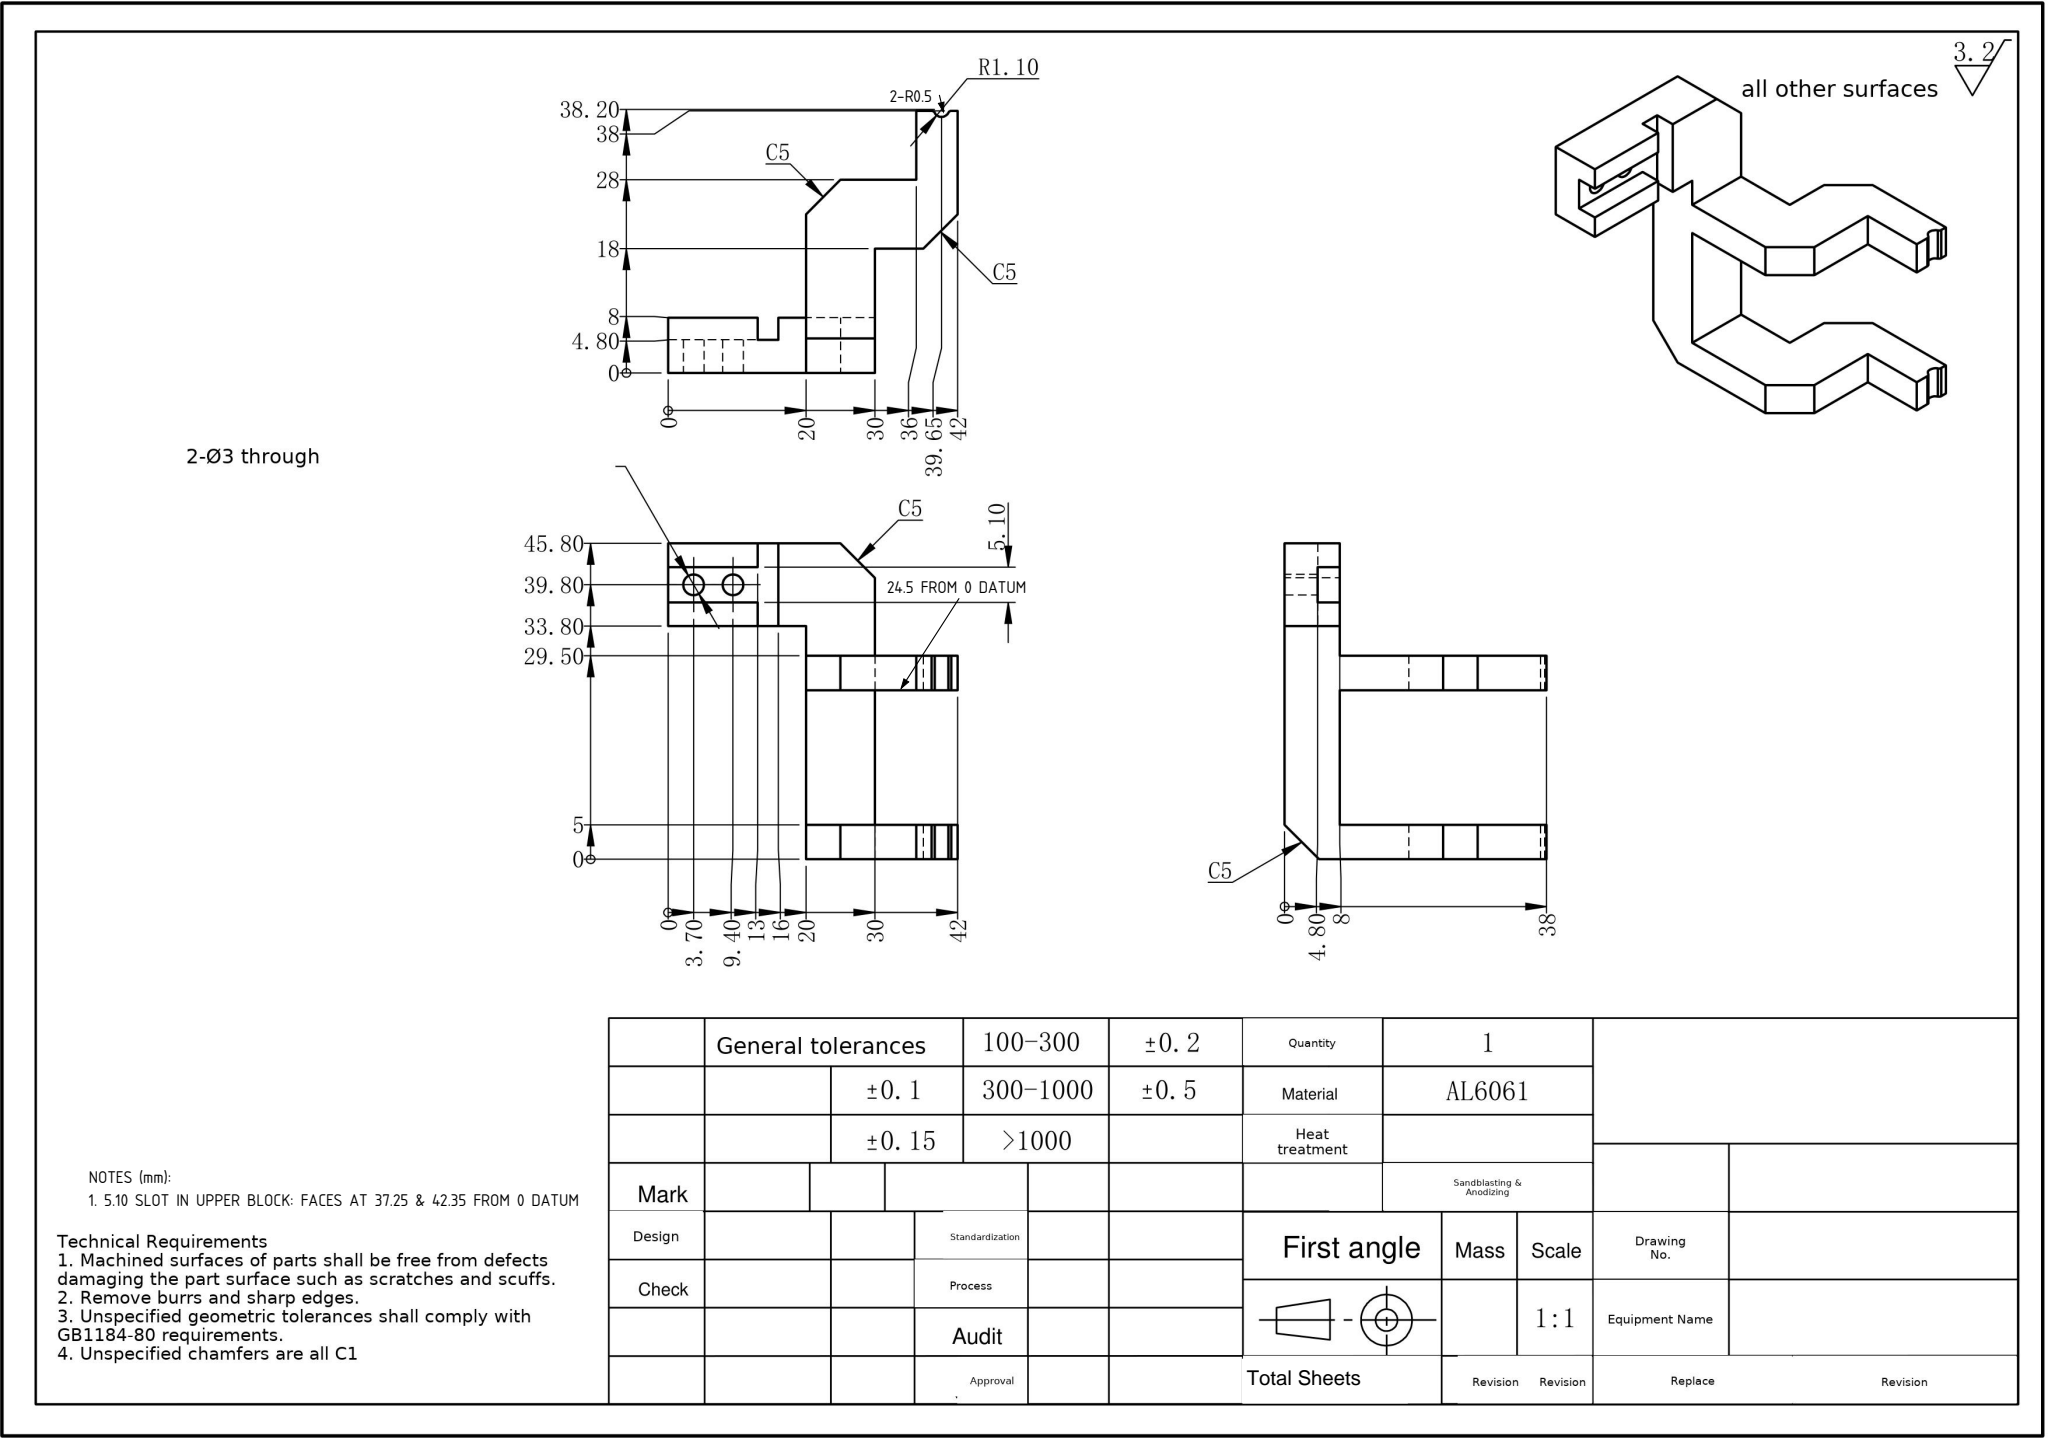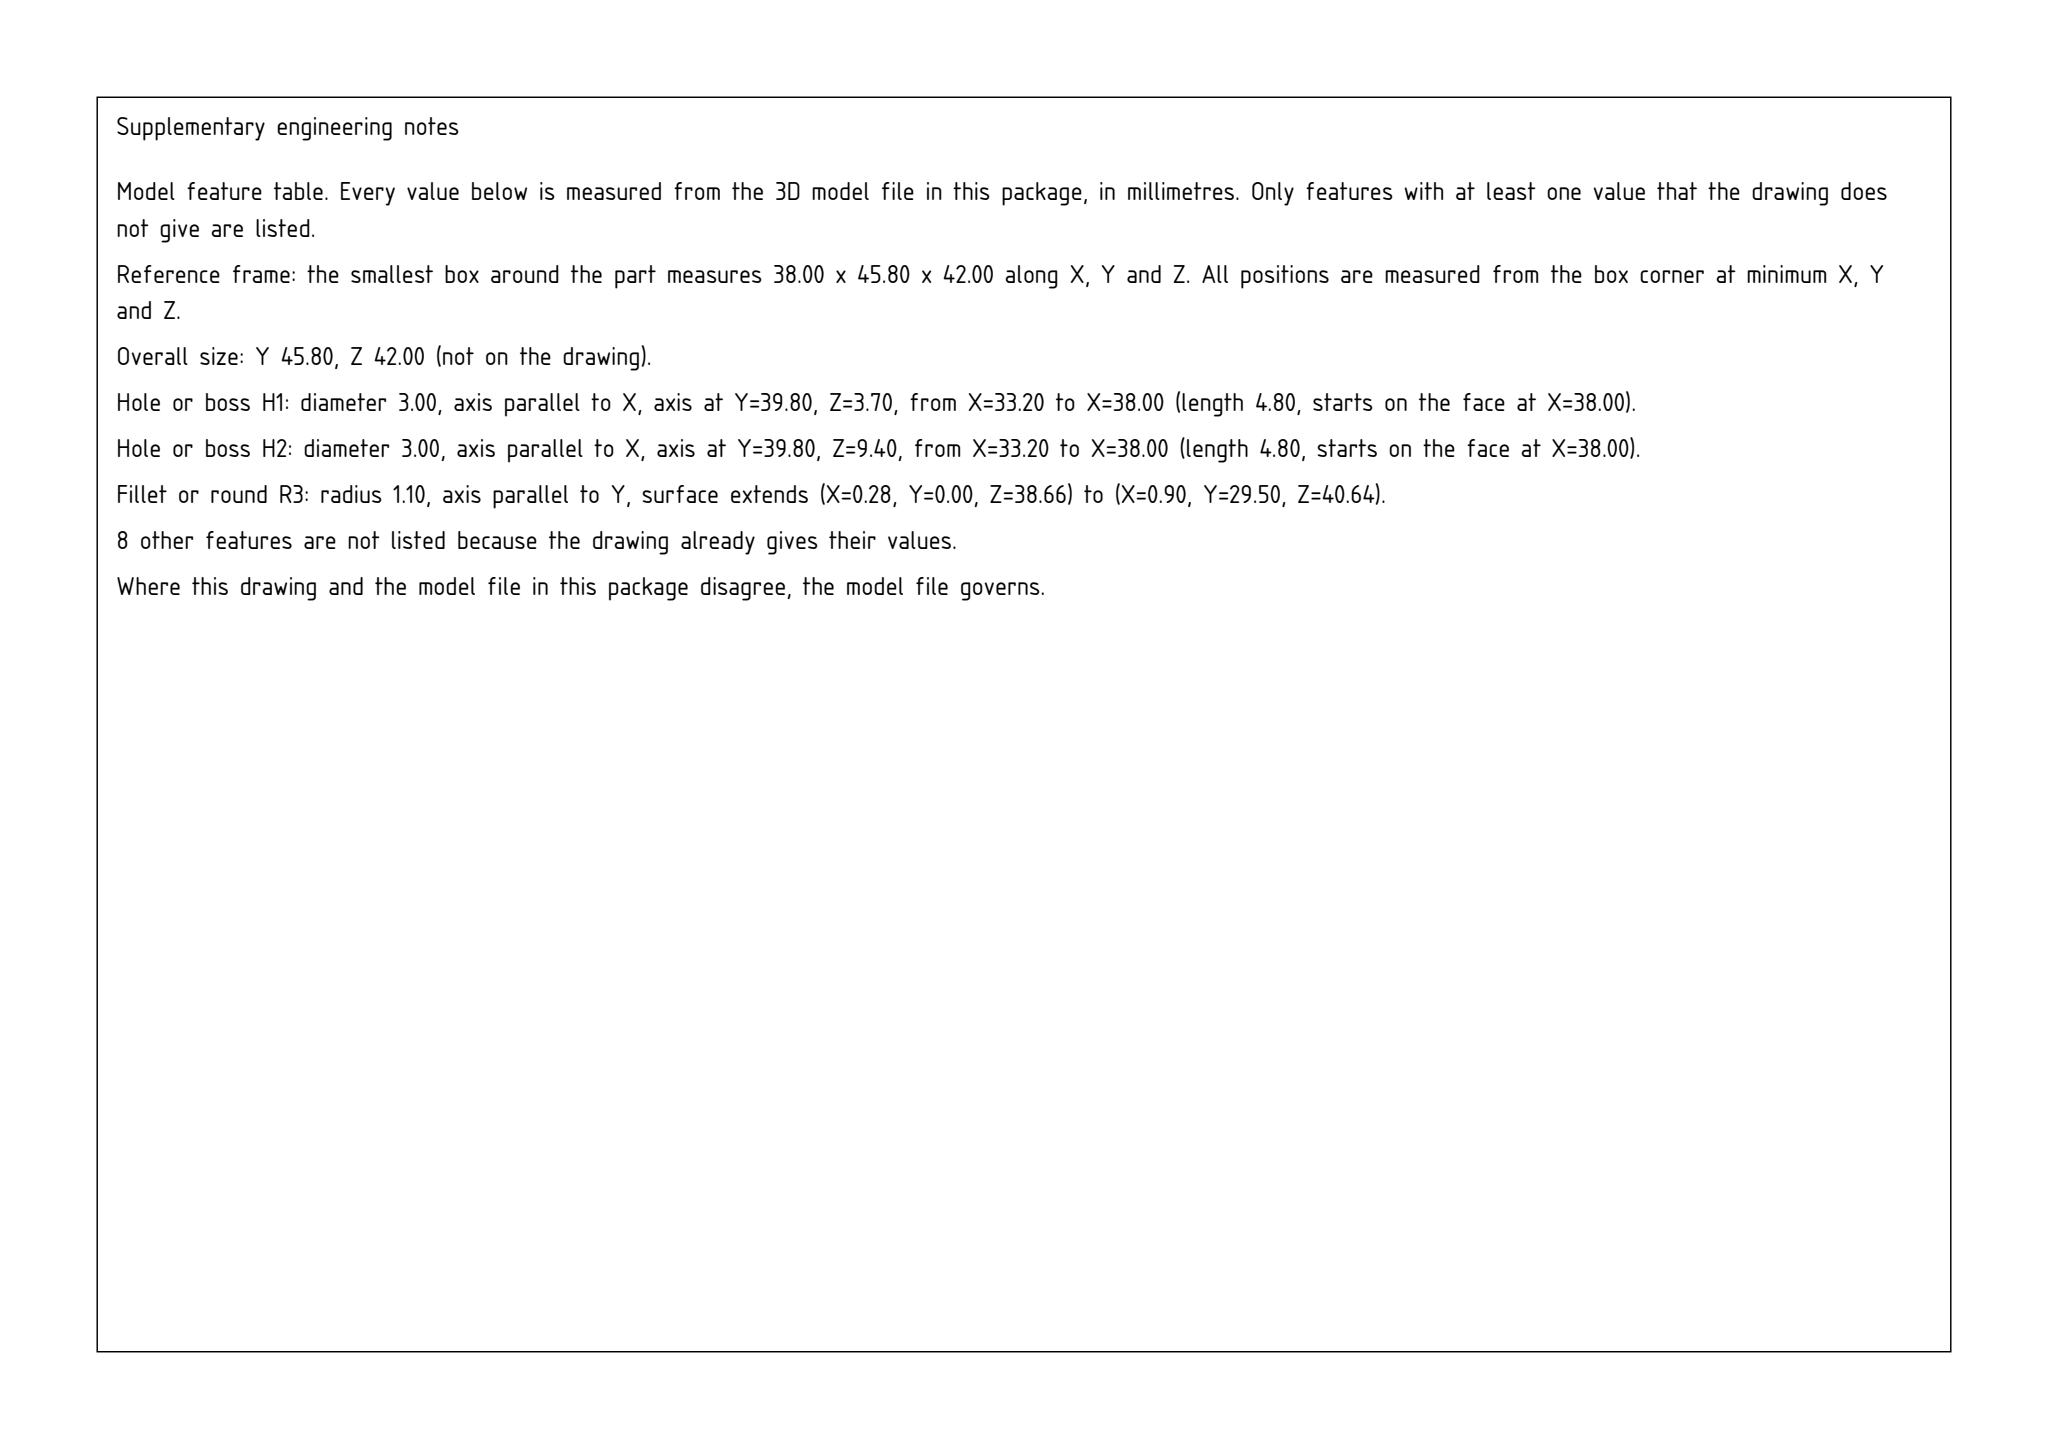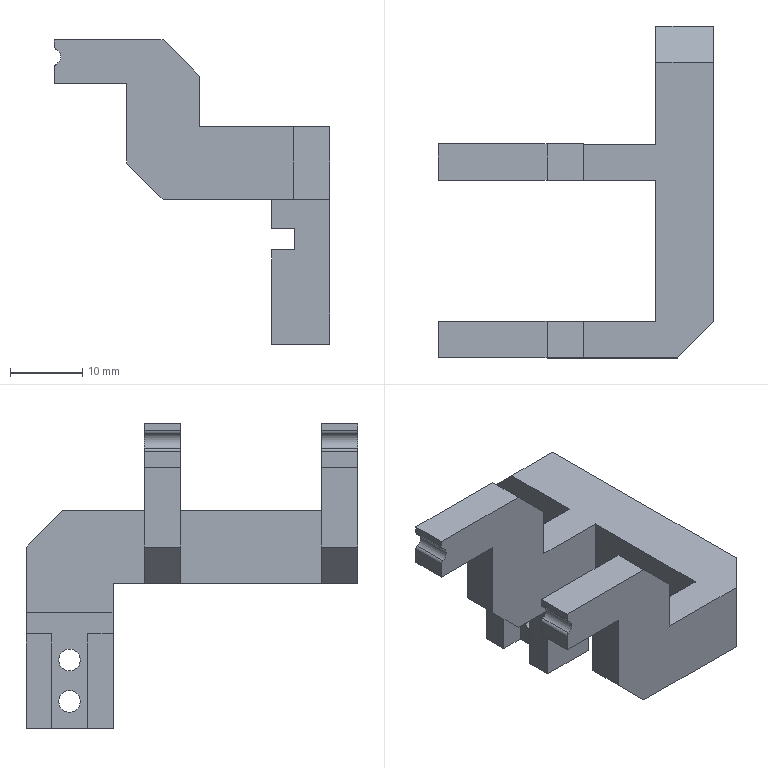Part | SolidWorks | mm | material AL6061 | 1 solid | 48 faces | box 38 x 45.8 x 42 mm | volume 8499 mm3 | plane 38 | cylinder 10 | commonest cylinder face diameters 3 x4 1 x4 2.2 x2
Drawing notes:
5.10 SLOT IN UPPER BLOCK: FACES AT 37.25 & 42.35 FROM 0 DATUM | from the solid: y-planes at 37.25 and 42.35 (42.35-37.25=5.10 slot width), y datum 0 = bbox min face
UPPER FORK ARM INNER FACE 24.5 FROM 0 DATUM; ARM 5 THK, GAP 19.5 | from the solid: y-planes 24.5 and 29.5 (arm 5 thk); lower arm face y=5 -> clear gap 24.5-5=19.5
2-R0.5 (2-Ø1) AT R1.10 NOTCH MOUTH: X 37.5, Z 38.21 & 41.09 | from the solid: Ø1 cyl, axis y, at step x=0.5 (=38-0.5=37.5 drawing X), z=38.21 and z=41.09, len 5, qty 2 each
build123d program:
from build123d import *

# Parameters (mm, degrees)
SKETCH1_W           = 8
SKETCH1_H           = 30
BOSS_EXTRUDE1_DEPTH = 6
SKETCH2_W           = 32
SKETCH2_H           = 5.1
CUT_EXTRUDE1_DEPTH  = 2.2
SKETCH3_W           = 3
SKETCH3_H           = 12
CUT_EXTRUDE2_DEPTH  = 2.2
SKETCH4_R           = 1.5
CUT_EXTRUDE3_DEPTH  = 10
SKETCH5_W           = 8
SKETCH5_H           = 10
BOSS_EXTRUDE2_DEPTH = 33.8
SKETCH6_W           = 10
SKETCH6_H           = 5
BOSS_EXTRUDE3_DEPTH = 30
SKETCH7_W           = 20
SKETCH7_H           = 5
BOSS_EXTRUDE4_DEPTH = 12
SKETCH8_W           = 10
SKETCH8_H           = 16
CUT_EXTRUDE4_DEPTH  = 12
SKETCH9_R           = 1.1
CUT_EXTRUDE5_DEPTH  = 64.108
FILLET1_R           = 0.5
SKETCH10_W          = 10
SKETCH10_H          = 5
BOSS_EXTRUDE5_DEPTH = 30
SKETCH11_W          = 20
SKETCH11_H          = 5
BOSS_EXTRUDE6_DEPTH = 12
CUT_EXTRUDE6_DEPTH  = 10
CHAMFER1_SIZE       = 5
MOVE_FACE1_BY       = 1


with BuildPart() as part:
    # Sketch1 → Boss-Extrude1 (new, symmetric)
    with BuildSketch(Plane(origin=(0, 0, 0), x_dir=(1, 0, 0), z_dir=(0, 1, 0))):
        Rectangle(SKETCH1_W, SKETCH1_H)
    extrude(amount=BOSS_EXTRUDE1_DEPTH, both=True)

    # Sketch2 → Cut-Extrude1 (cut)
    with BuildSketch(Plane.ZY.offset(4)):
        with Locations((-15, 0)):
            Rectangle(SKETCH2_W, SKETCH2_H)
    extrude(amount=-CUT_EXTRUDE1_DEPTH, mode=Mode.SUBTRACT)

    # Sketch3 → Cut-Extrude2 (cut)
    with BuildSketch(Plane.ZY.offset(4)):
        with Locations((-0.5, 0)):
            Rectangle(SKETCH3_W, SKETCH3_H)
    extrude(amount=-CUT_EXTRUDE2_DEPTH, mode=Mode.SUBTRACT)

    # Sketch4 → Cut-Extrude3 (cut)
    with BuildSketch(Plane(origin=(4, 0, 0), x_dir=(0, 0, -1), z_dir=(1, 0, 0))):
        with Locations((11.3, 0)):
            Circle(SKETCH4_R)
        with Locations((5.6, 0)):
            Circle(SKETCH4_R)
    extrude(amount=-CUT_EXTRUDE3_DEPTH, mode=Mode.SUBTRACT)

    # Sketch5 → Boss-Extrude2 (add)
    with BuildSketch(Plane.XZ.offset(6)):
        with Locations((0, 10)):
            Rectangle(SKETCH5_W, SKETCH5_H)
    extrude(amount=BOSS_EXTRUDE2_DEPTH)

    # Sketch6 → Boss-Extrude3 (add)
    with BuildSketch(Plane.ZY.offset(4)):
        with Locations((10, -37.3)):
            Rectangle(SKETCH6_W, SKETCH6_H)
    extrude(amount=BOSS_EXTRUDE3_DEPTH)

    # Sketch7 → Boss-Extrude4 (add)
    with BuildSketch(Plane.XY.offset(15)):
        with Locations((-24, -37.3)):
            Rectangle(SKETCH7_W, SKETCH7_H)
    extrude(amount=BOSS_EXTRUDE4_DEPTH)

    # Sketch8 → Cut-Extrude4 (cut)
    with BuildSketch(Plane.XZ.offset(39.8)):
        with Locations((-29, 13)):
            Rectangle(SKETCH8_W, SKETCH8_H)
    extrude(amount=-CUT_EXTRUDE4_DEPTH, mode=Mode.SUBTRACT)

    # Sketch9 → Cut-Extrude5 (cut, through all)
    with BuildSketch(Plane.XZ.offset(39.8)):
        with Locations((-34.2, 24.648)):
            Circle(SKETCH9_R)
    extrude(amount=-CUT_EXTRUDE5_DEPTH, mode=Mode.SUBTRACT)

    # Fillet1
    fillet1_edges = [part.edges().sort_by_distance(p)[0] for p in [
        (-34, -37.3, 25.73),
        (-34, -37.3, 23.567),
    ]]
    fillet(fillet1_edges, radius=FILLET1_R)

    # Sketch10 → Boss-Extrude5 (add)
    with BuildSketch(Plane.ZY.offset(4)):
        with Locations((10, -12.8)):
            Rectangle(SKETCH10_W, SKETCH10_H)
    extrude(amount=BOSS_EXTRUDE5_DEPTH)

    # Sketch11 → Boss-Extrude6 (add)
    with BuildSketch(Plane.XY.offset(15)):
        with Locations((-24, -12.8)):
            Rectangle(SKETCH11_W, SKETCH11_H)
    extrude(amount=BOSS_EXTRUDE6_DEPTH)

    # Sketch12 → Cut-Extrude6 (cut)
    with BuildSketch(Plane.XZ.offset(15.3)):
        with BuildLine():
            Line((-24, 21), (-34, 21))
            Line((-34, 21), (-34, 23.21))
            ThreePointArc((-34, 23.21), (-33.924, 23.475), (-33.719, 23.659))
            ThreePointArc((-33.719, 23.659), (-33.1, 24.648), (-33.719, 25.638))
            ThreePointArc((-33.719, 25.638), (-33.924, 25.822), (-34, 26.087))
            Line((-34, 26.087), (-36.341, 26.087))
            Line((-36.341, 26.087), (-36.341, -0.6034))
            Line((-36.341, -0.6034), (-24, -1.068))
            Line((-24, -1.068), (-24, 5))
            Line((-24, 5), (-24, 21))
        make_face()
    extrude(amount=-CUT_EXTRUDE6_DEPTH, mode=Mode.SUBTRACT)

    # Chamfer1
    chamfer1_edges = [part.edges().sort_by_distance(p)[0] for p in [
        (-14, -37.3, 27),
        (-24, -37.3, 5),
        (0, 6, 15),
        (-14, -12.8, 27),
        (-24, -12.8, 5),
        (4, -39.8, 10),
    ]]
    chamfer(chamfer1_edges, length=CHAMFER1_SIZE)

    # Move Face1: a face moved inward by 1.0
    extrude(part.faces().sort_by_distance((-1.8, 0, -3))[0], amount=MOVE_FACE1_BY, dir=(1, 0, 0), mode=Mode.SUBTRACT)


solid = part.part